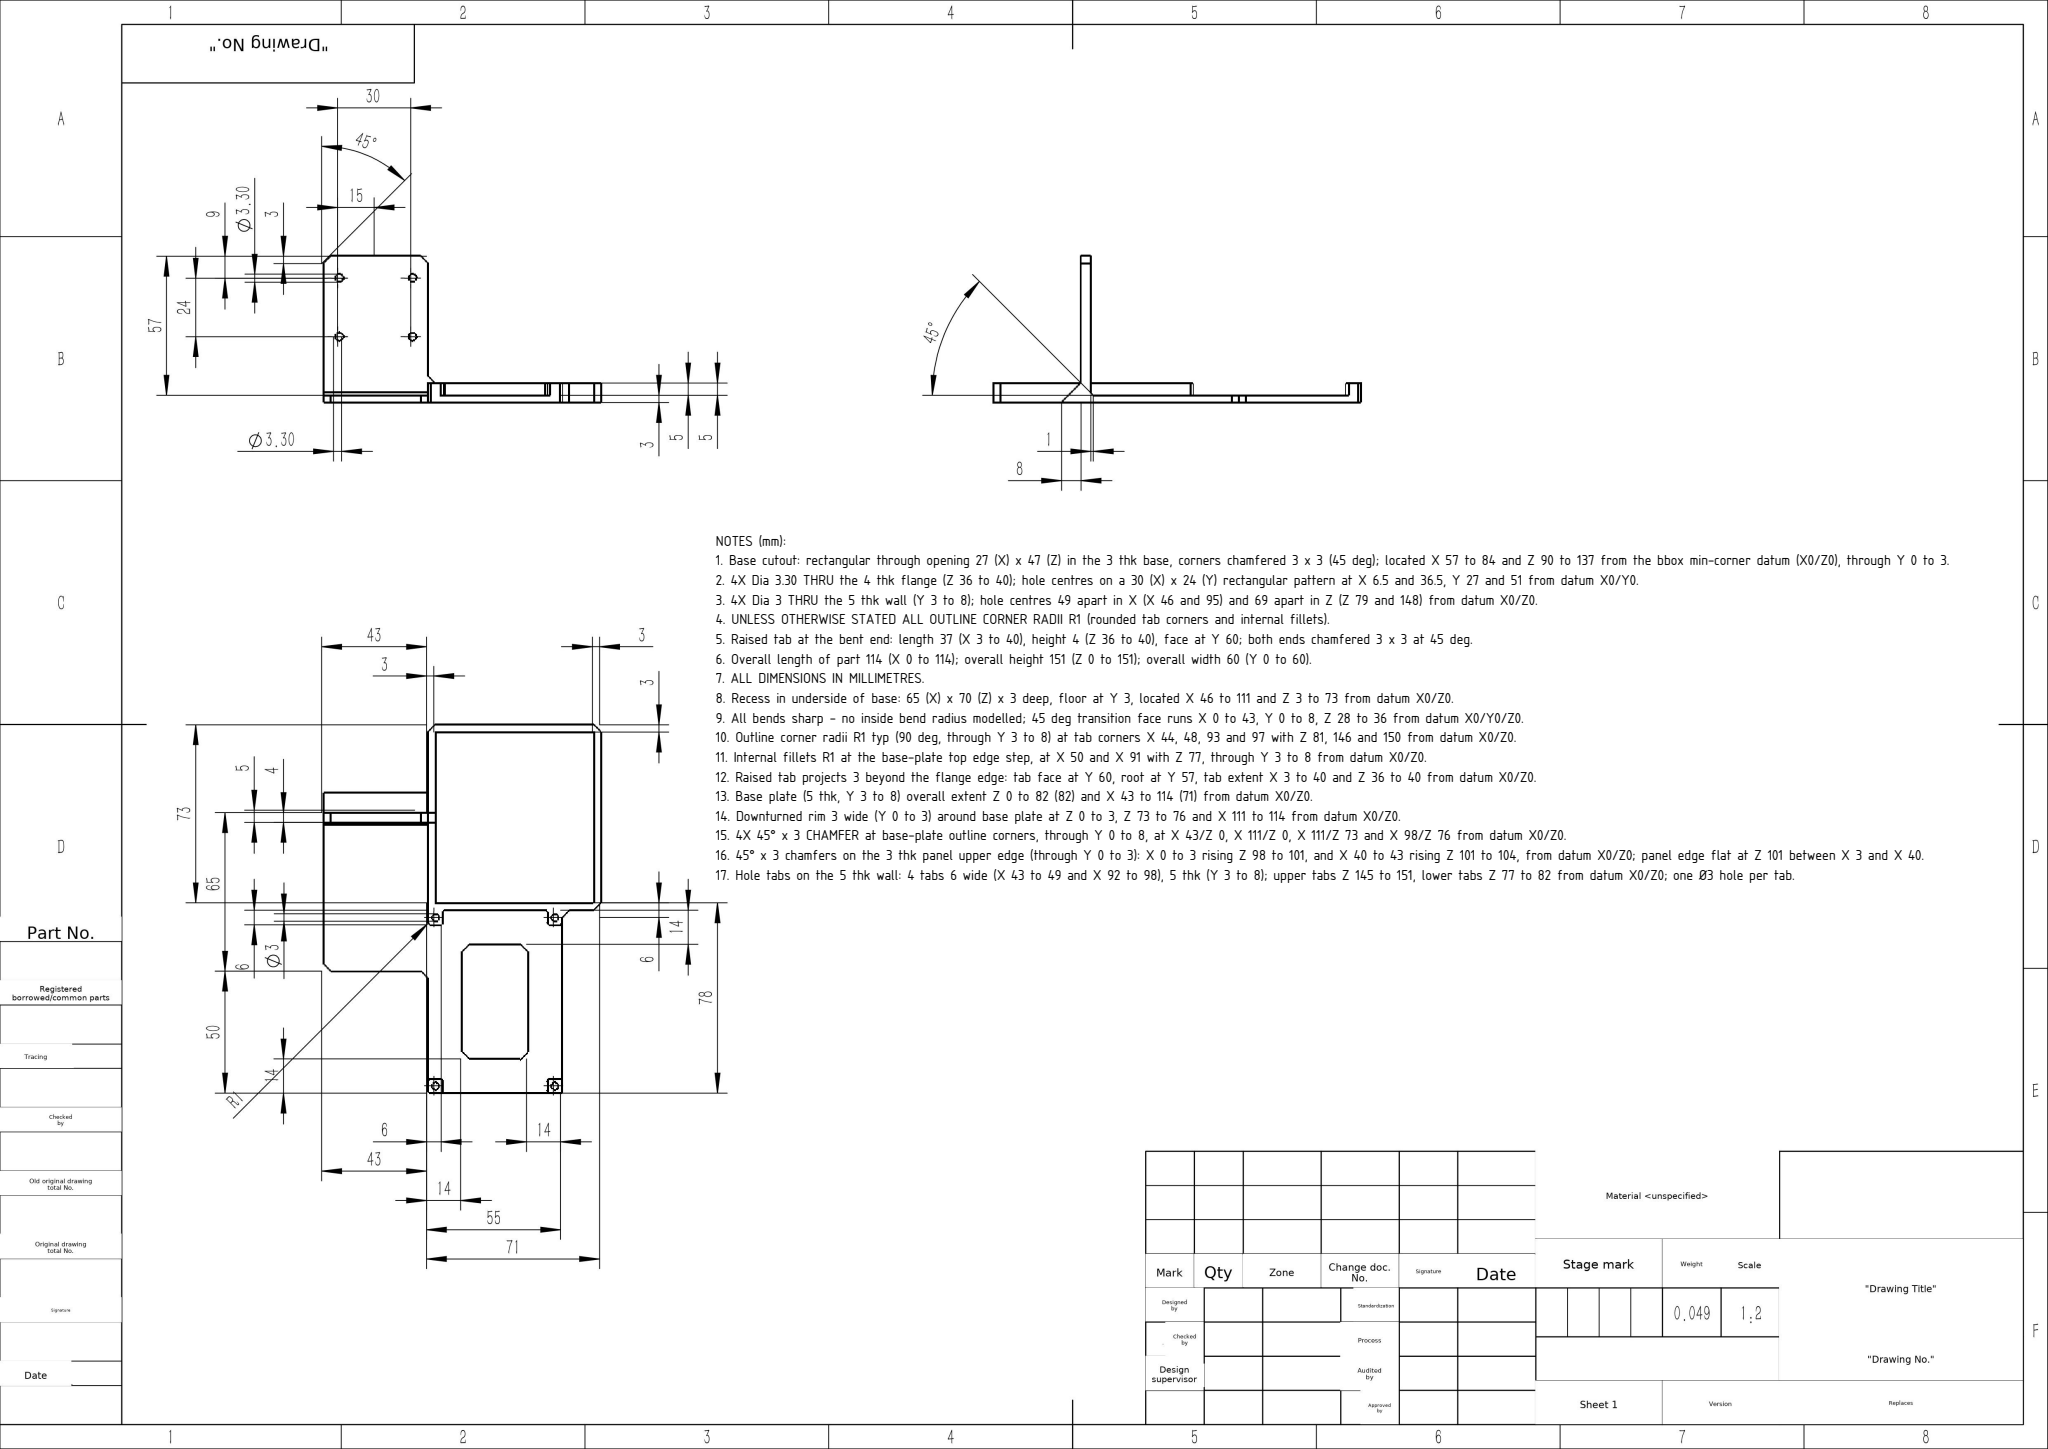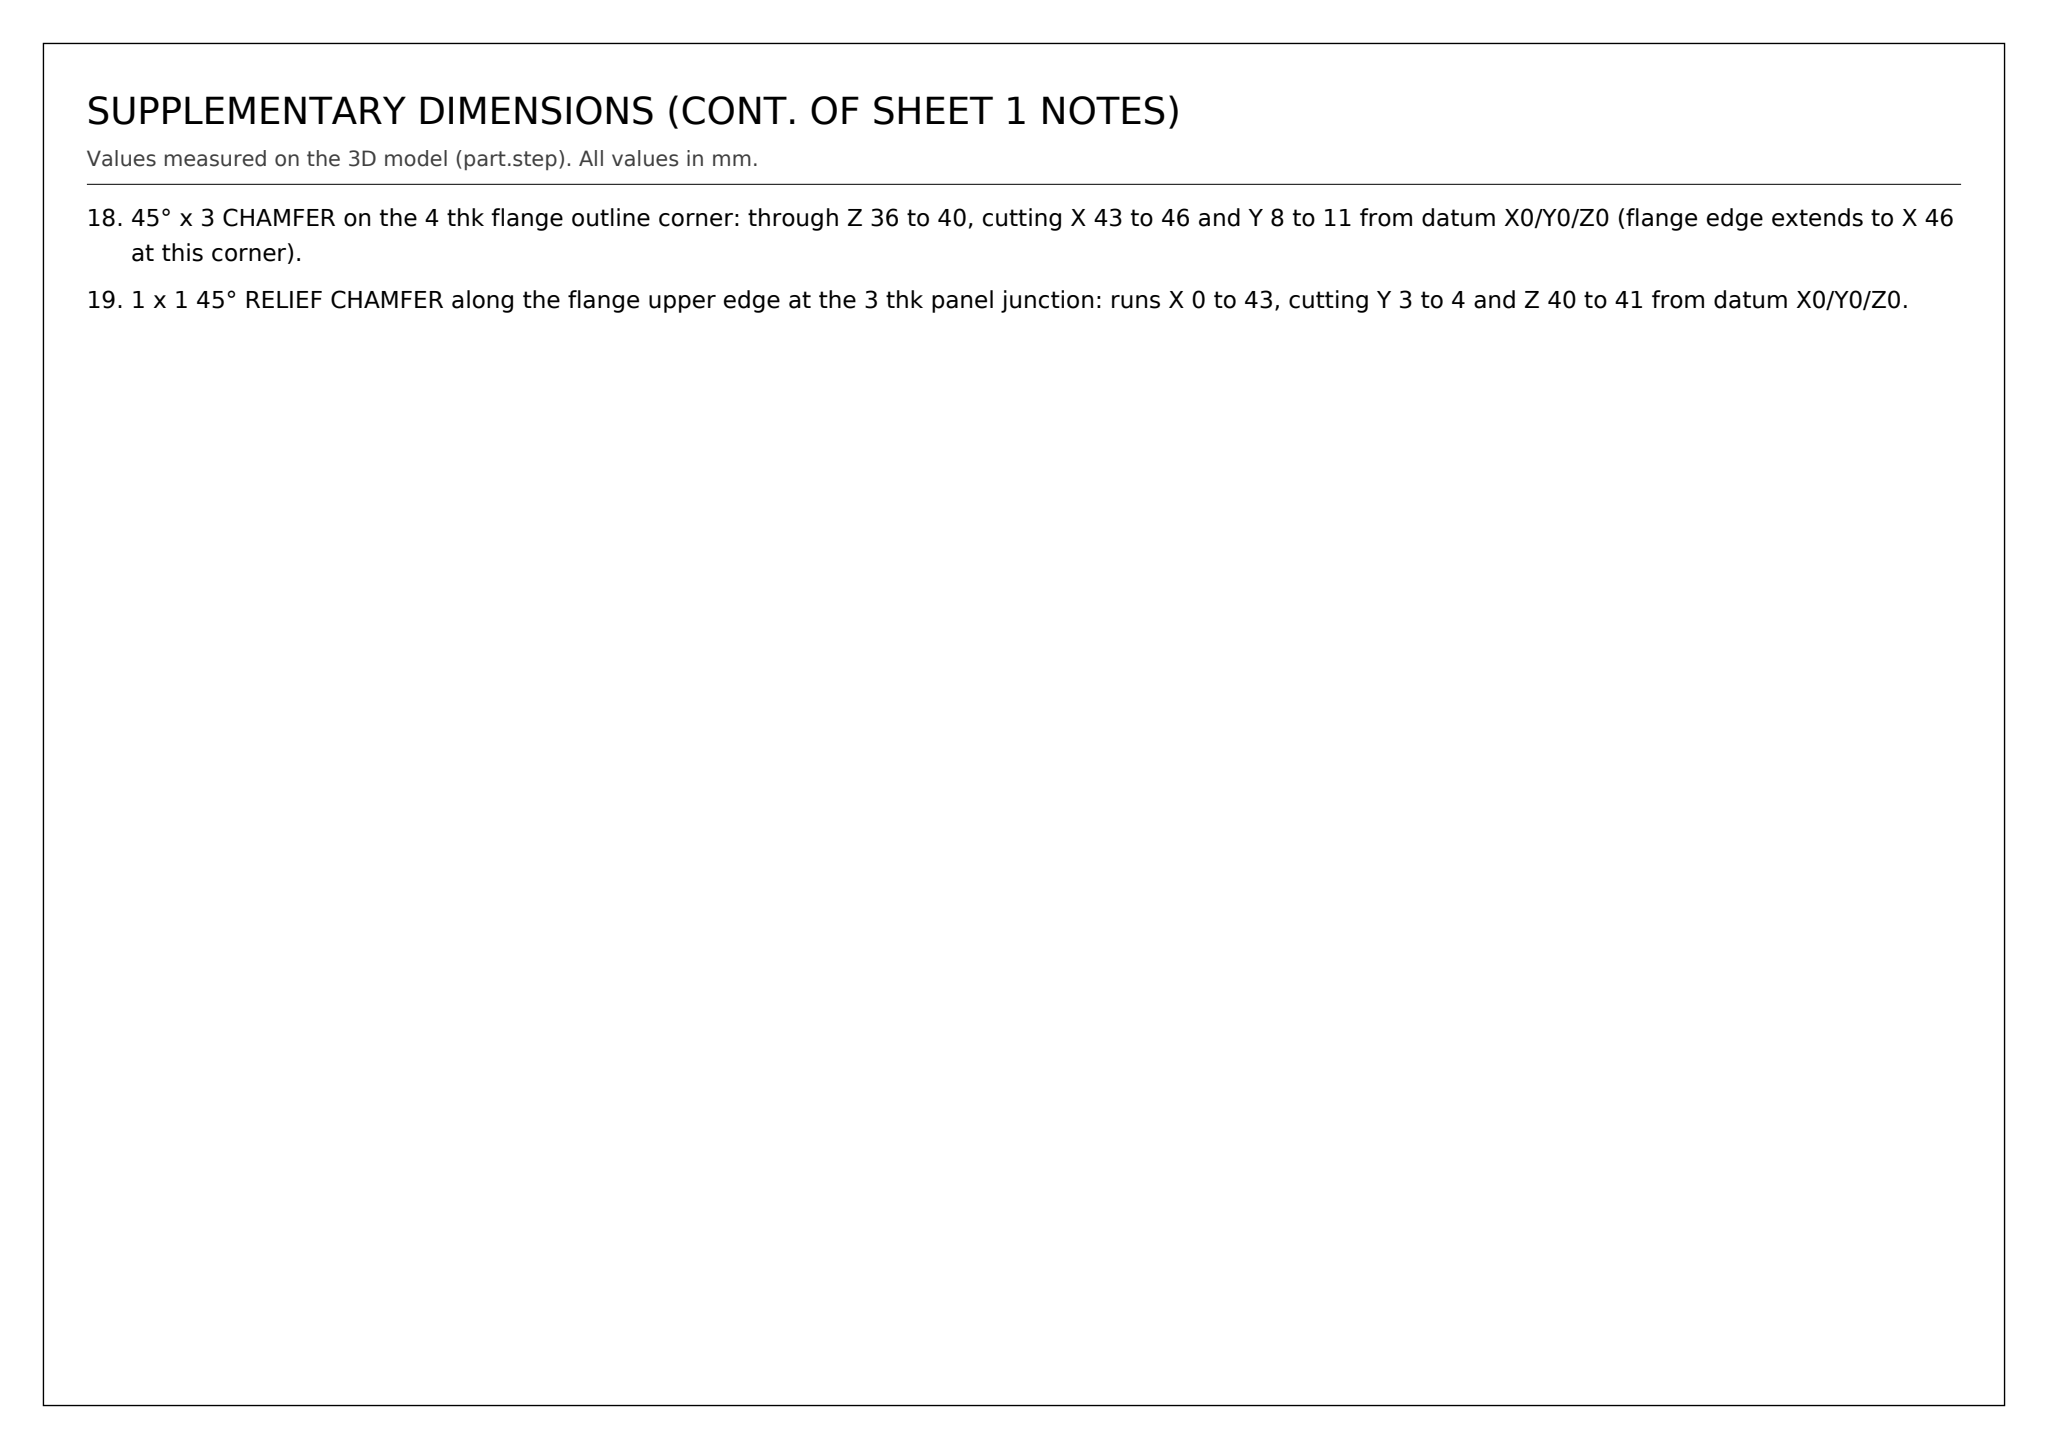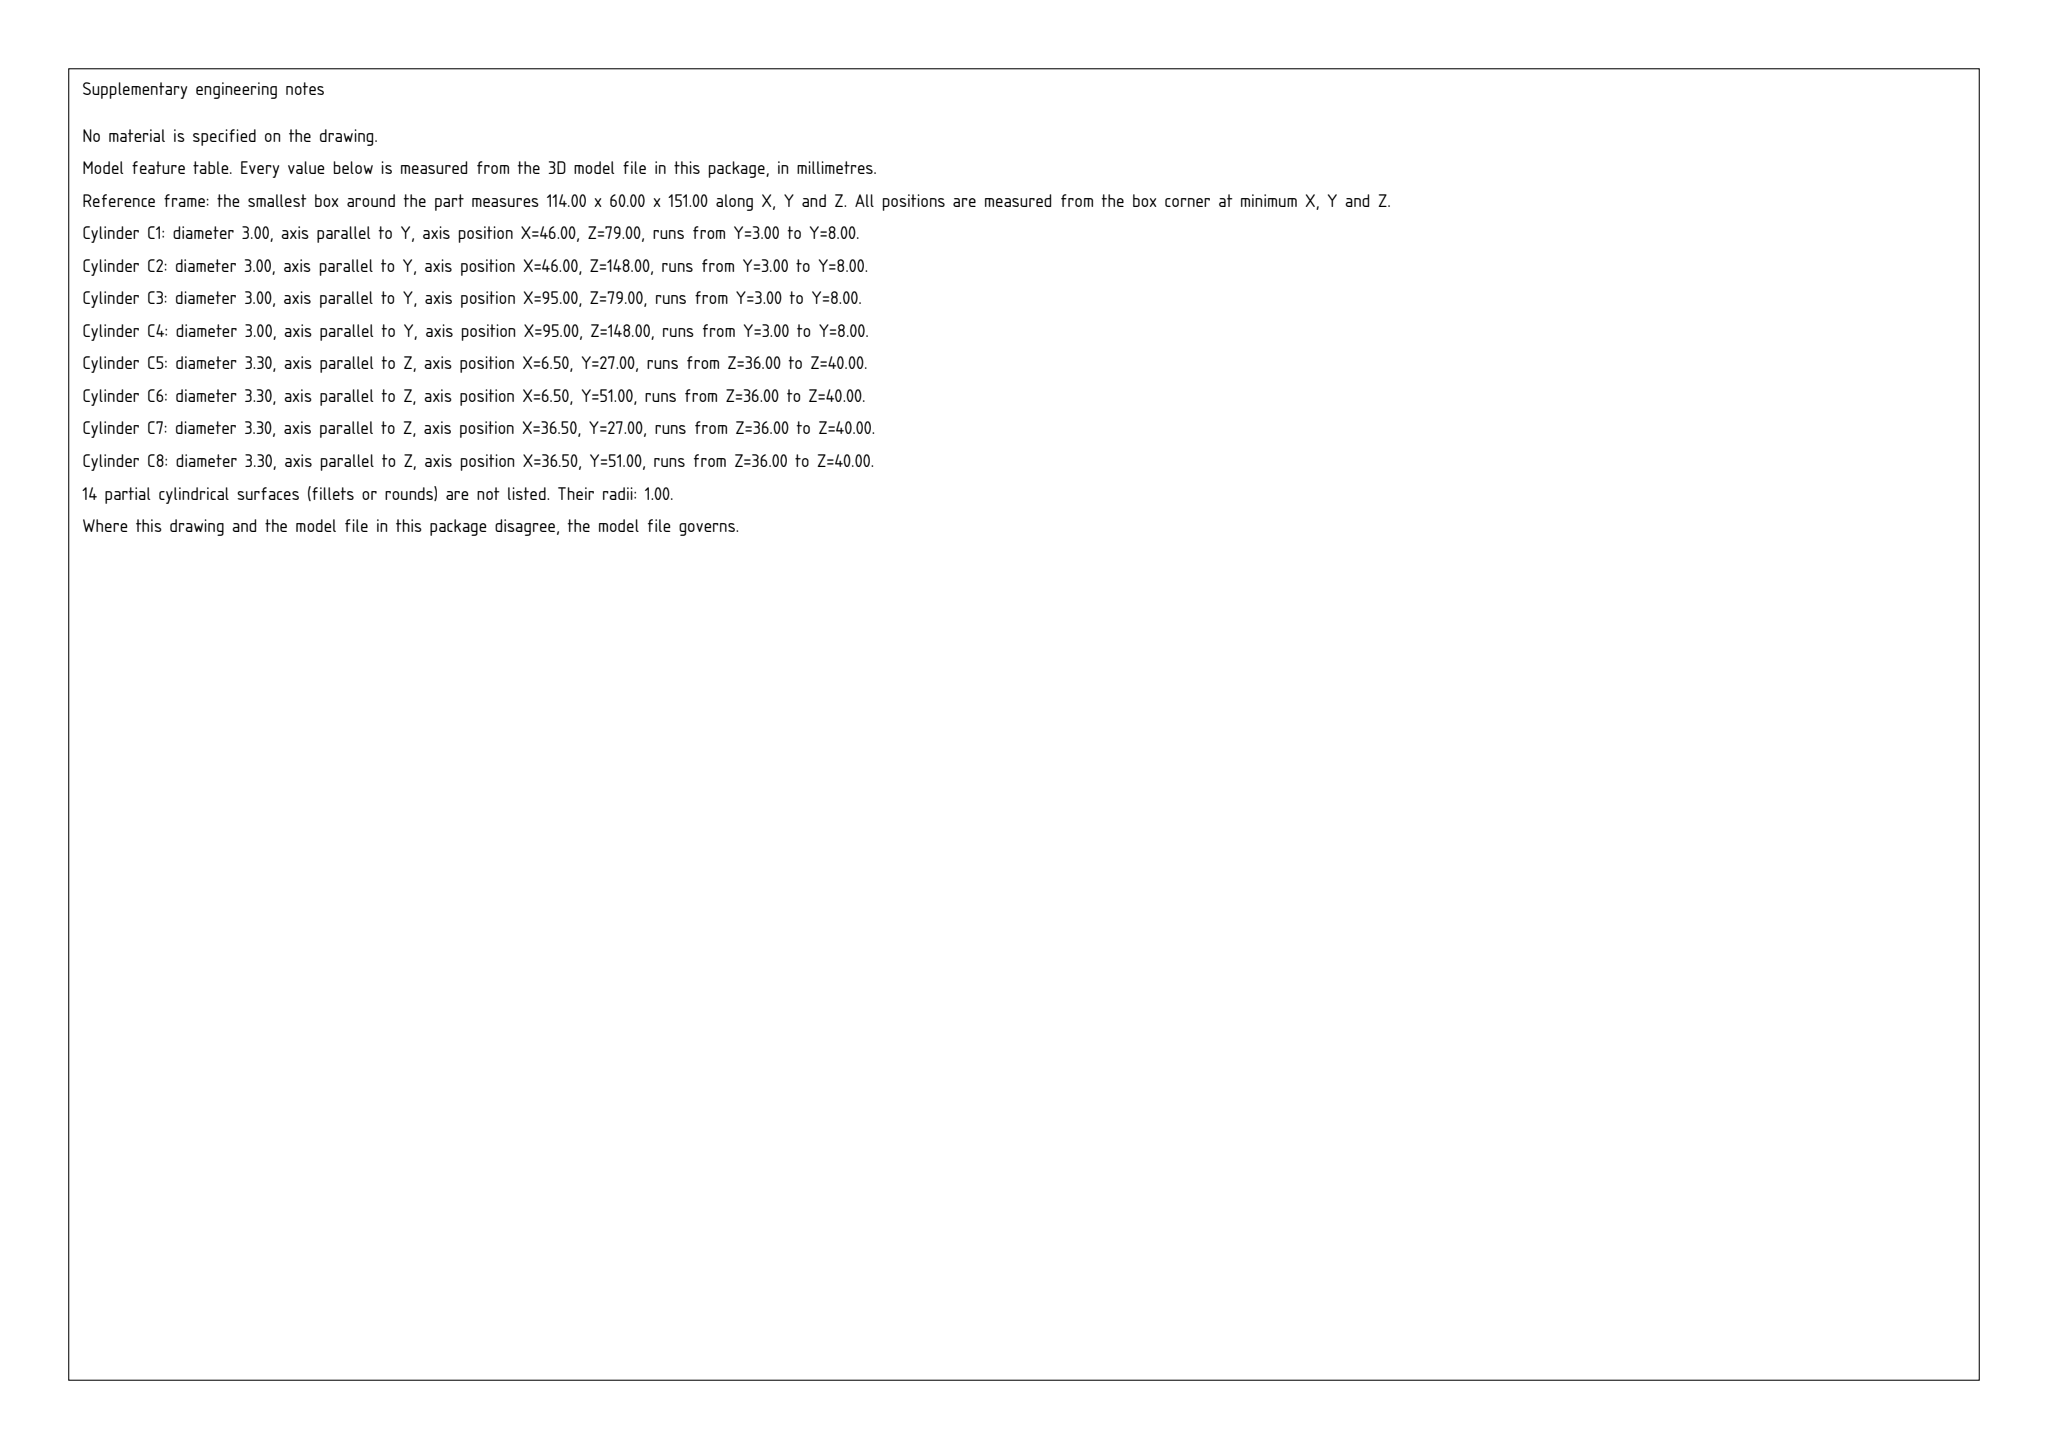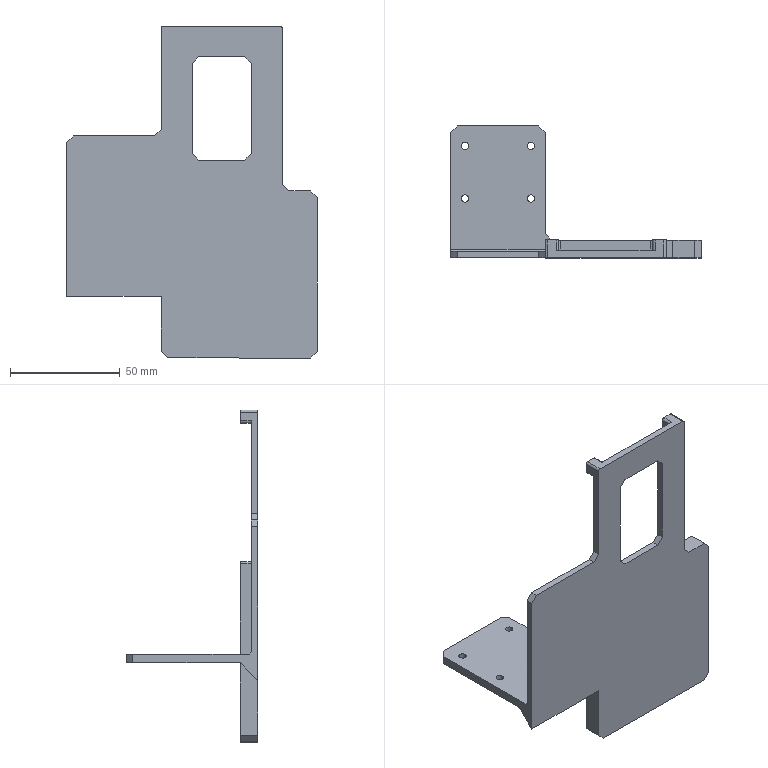Part | SolidWorks | mm | 1 solid | 86 faces | box 114 x 60 x 151 mm | volume 48966 mm3 | plane 56 | cylinder 30 | commonest cylinder face diameters 2 x14 3.3 x8 3 x8
Drawing notes:
Base cutout: rectangular through opening 27 (X) x 47 (Z) in the 3 thk base, corners chamfered 3 x 3 (45 deg); located X 57 to 84 and Z 90 to 137 from the bbox min-corner datum (X0/Z0), through Y 0 to 3. | from the solid: axis_planes x=57 and x=84 (y 0-3, z 93-134); z=90 and z=137 planes (x 60-81, y 0-3); four inclined 45 deg planes 3x3x3 at (57,0,90),(57,0,134),(81,0,90),(81,0,134)
4X Dia 3.30 THRU the 4 thk flange (Z 36 to 40); hole centres on a 30 (X) x 24 (Y) rectangular pattern at X 6.5 and 36.5, Y 27 and 51 from datum X0/Y0. | from the solid: cylinders hole/bore dia 3.3 axis z at (6.5,27),(6.5,51),(36.5,27),(36.5,51), from 36 to 40
4X Dia 3 THRU the 5 thk wall (Y 3 to 8); hole centres 49 apart in X (X 46 and 95) and 69 apart in Z (Z 79 and 148) from datum X0/Z0. | from the solid: cylinders hole/bore dia 3.0 axis y at (46,148),(46,79),(95,148),(95,79), from 3 to 8
UNLESS OTHERWISE STATED ALL OUTLINE CORNER RADII R1 (rounded tab corners and internal fillets). | from the solid: convex arcs dia 2.0 at (44/48/93/97, z 81/146/150) and concave arcs dia 2.0 at (50,77) and (91,77) -> R1
Raised tab at the bent end: length 37 (X 3 to 40), height 4 (Z 36 to 40), face at Y 60; both ends chamfered 3 x 3 at 45 deg. | from the solid: axis_plane y=60 extent x 3-40, z 36-40 (area 148); inclined planes [45,45,90] at (0,57,36) and (40,57,36) size 3x3x4
Overall length of part 114 (X 0 to 114); overall height 151 (Z 0 to 151); overall width 60 (Y 0 to 60). | from the solid: bbox_xyz [114.0, 60.0, 151.0]
ALL DIMENSIONS IN MILLIMETRES. | from the solid: STEP model facts stated in mm
Recess in underside of base: 65 (X) x 70 (Z) x 3 deep, floor at Y 3, located X 46 to 111 and Z 3 to 73 from datum X0/Z0. | from the solid: plane y=3 extent x[46,111] z[3,73] area 4550; bounding faces x=46 and x=111 (y 3-8, z 3-73) and z=3 and z=73 (x 46-111, y 3-8)
All bends sharp - no inside bend radius modelled; 45 deg transition face runs X 0 to 43, Y 0 to 8, Z 28 to 36 from datum X0/Y0/Z0. | from the solid: tori[minor_r,major_r] list empty; inclined plane angle_to_xyz [90,45,45] bbox_from [0,0,28] size [43,8,8]
Outline corner radii R1 typ (90 deg, through Y 3 to 8) at tab corners X 44, 48, 93 and 97 with Z 81, 146 and 150 from datum X0/Z0. | from the solid: convex arc (round/outer radius) dia 2.0 axis y at (44,81),(48,81),(93,81),(97,81),(44,146),(48,146),(93,146),(97,146),(44,150),(48,150),(93,150),(97,150)
Internal fillets R1 at the base-plate top edge step, at X 50 and X 91 with Z 77, through Y 3 to 8 from datum X0/Z0. | from the solid: concave arc (fillet) dia 2.0 axis y at (50,77) and (91,77), from y 3 to 8
Raised tab projects 3 beyond the flange edge: tab face at Y 60, root at Y 57, tab extent X 3 to 40 and Z 36 to 40 from datum X0/Z0. | from the solid: plane y=60 extent x[3,40] z[36,40]; inclined planes bbox_from [0,57,36] and [40,57,36] size [3,3,4]
Base plate (5 thk, Y 3 to 8) overall extent Z 0 to 82 (82) and X 43 to 114 (71) from datum X0/Z0. | from the solid: plane y=8 extent x[43,114] z[0,82]
Downturned rim 3 wide (Y 0 to 3) around base plate at Z 0 to 3, Z 73 to 76 and X 111 to 114 from datum X0/Z0. | from the solid: planes z=0 (x 46-111, y 0-8), z=3 (x 46-111, y 3-8), z=76 (x 101-111, y 0-8), x=114 (y 0-8, z 3-73), x=111 (y 3-8, z 3-73)
4X 45° x 3 CHAMFER at base-plate outline corners, through Y 0 to 8, at X 43/Z 0, X 111/Z 0, X 111/Z 73 and X 98/Z 76 from datum X0/Z0. | from the solid: inclined_planes: [45,90,45] bbox_from [43,0,0], [111,0,0], [111,0,73], [98,0,76], each size 3 x 8 x 3
45° x 3 chamfers on the 3 thk panel upper edge (through Y 0 to 3): X 0 to 3 rising Z 98 to 101, and X 40 to 43 rising Z 101 to 104, from datum X0/Z0; panel edge flat at Z 101 between X 3 and X 40. | from the solid: inclined_planes [45,90,45] bbox_from [0,0,98] size 3x3x3 and bbox_from [40,0,101] size 3x3x3; plane z=101 extent x [3,40], y [0,3]
Hole tabs on the 5 thk wall: 4 tabs 6 wide (X 43 to 49 and X 92 to 98), 5 thk (Y 3 to 8); upper tabs Z 145 to 151, lower tabs Z 77 to 82 from datum X0/Z0; one Ø3 hole per tab. | from the solid: planes y=8 extent x [43,49] z [145,151] and x [92,98] z [145,151]; planes z=145 and z=82 extent x [44,48] and x [93,97], y [3,8]; planes x=49 and x=92 extent y [3,8] z [77,81]
45° x 3 CHAMFER on the 4 thk flange outline corner: through Z 36 to 40, cutting X 43 to 46 and Y 8 to 11 from datum X0/Y0/Z0 (flange edge extends to X 46 at this corner). | from the solid: inclined_planes: angle_to_xyz_axes [45,45,90], bbox_from [43.0,8.0,36.0], size [3,3,4]
1 x 1 45° RELIEF CHAMFER along the flange upper edge at the 3 thk panel junction: runs X 0 to 43, cutting Y 3 to 4 and Z 40 to 41 from datum X0/Y0/Z0. | from the solid: inclined_planes: angle_to_xyz_axes [90,45,45], bbox_from [0.0,3.0,40.0], size [43,1,1]